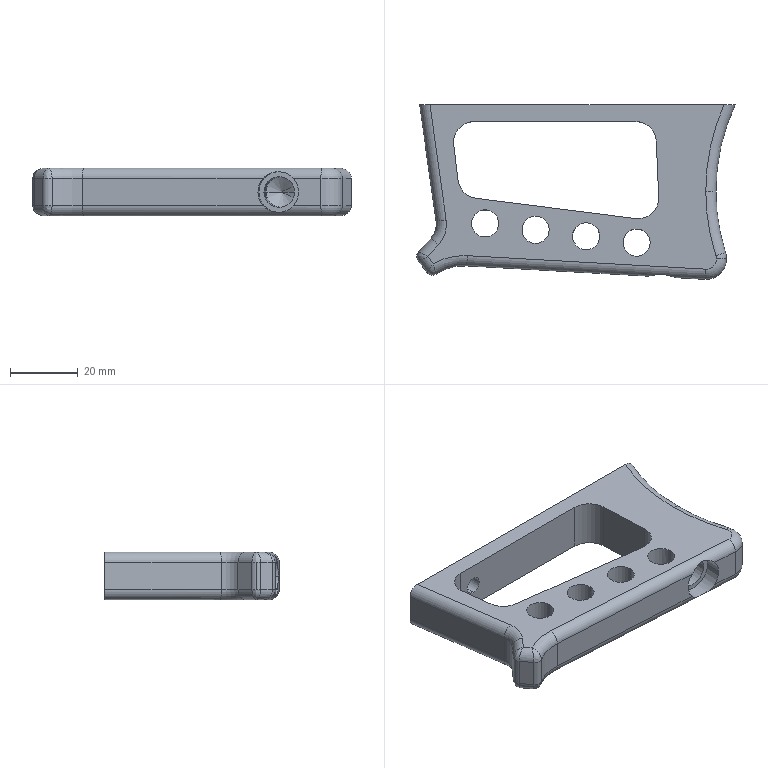Component | SolidWorks | Stock-1 | 1 solid | 70 faces | box 93.85 x 51.48 x 14 mm | volume 33996 mm3 | cylinder 37 | plane 13 | torus 12 | cone 4 | spline 4 | commonest cylinder face diameters 12 x9 8 x8 6 x8 5 x4 4 x3 9 x2 120 x2 30 x1